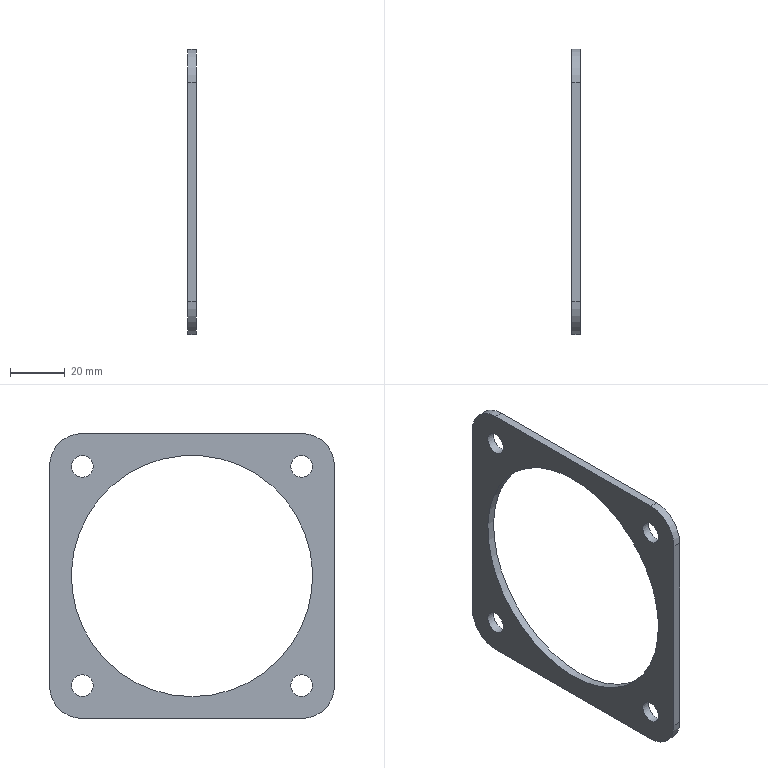Component | NX | GASKET | 1 solid | 15 faces | volume 13228 mm3 | cylinder 9 | plane 6 | commonest cylinder face diameters 8 x4 24 x4 88 x1